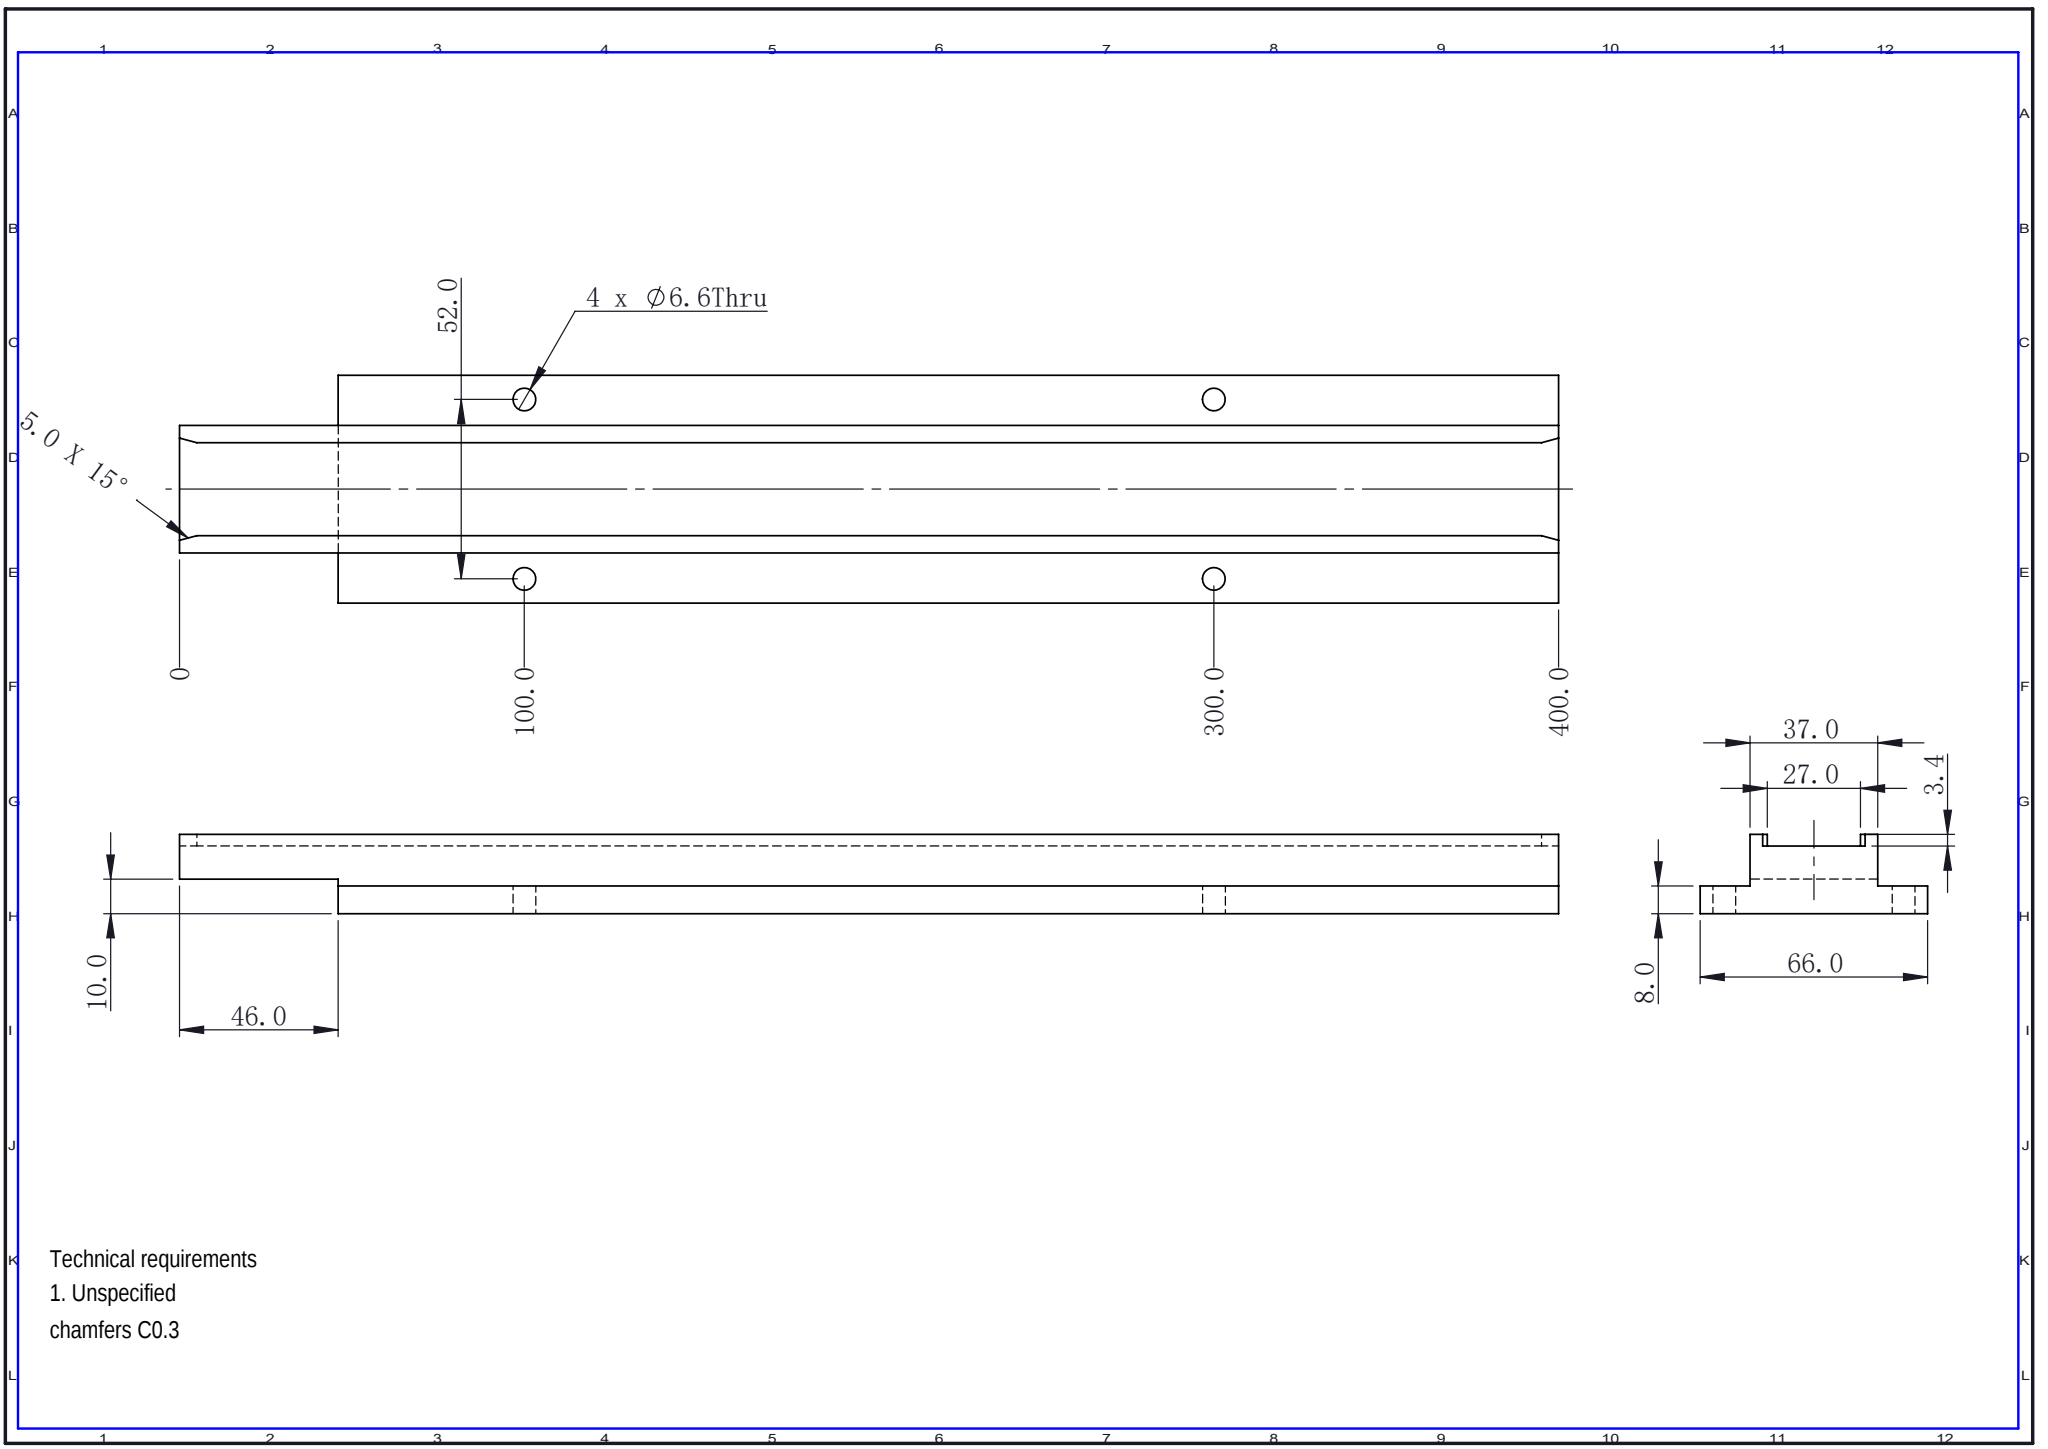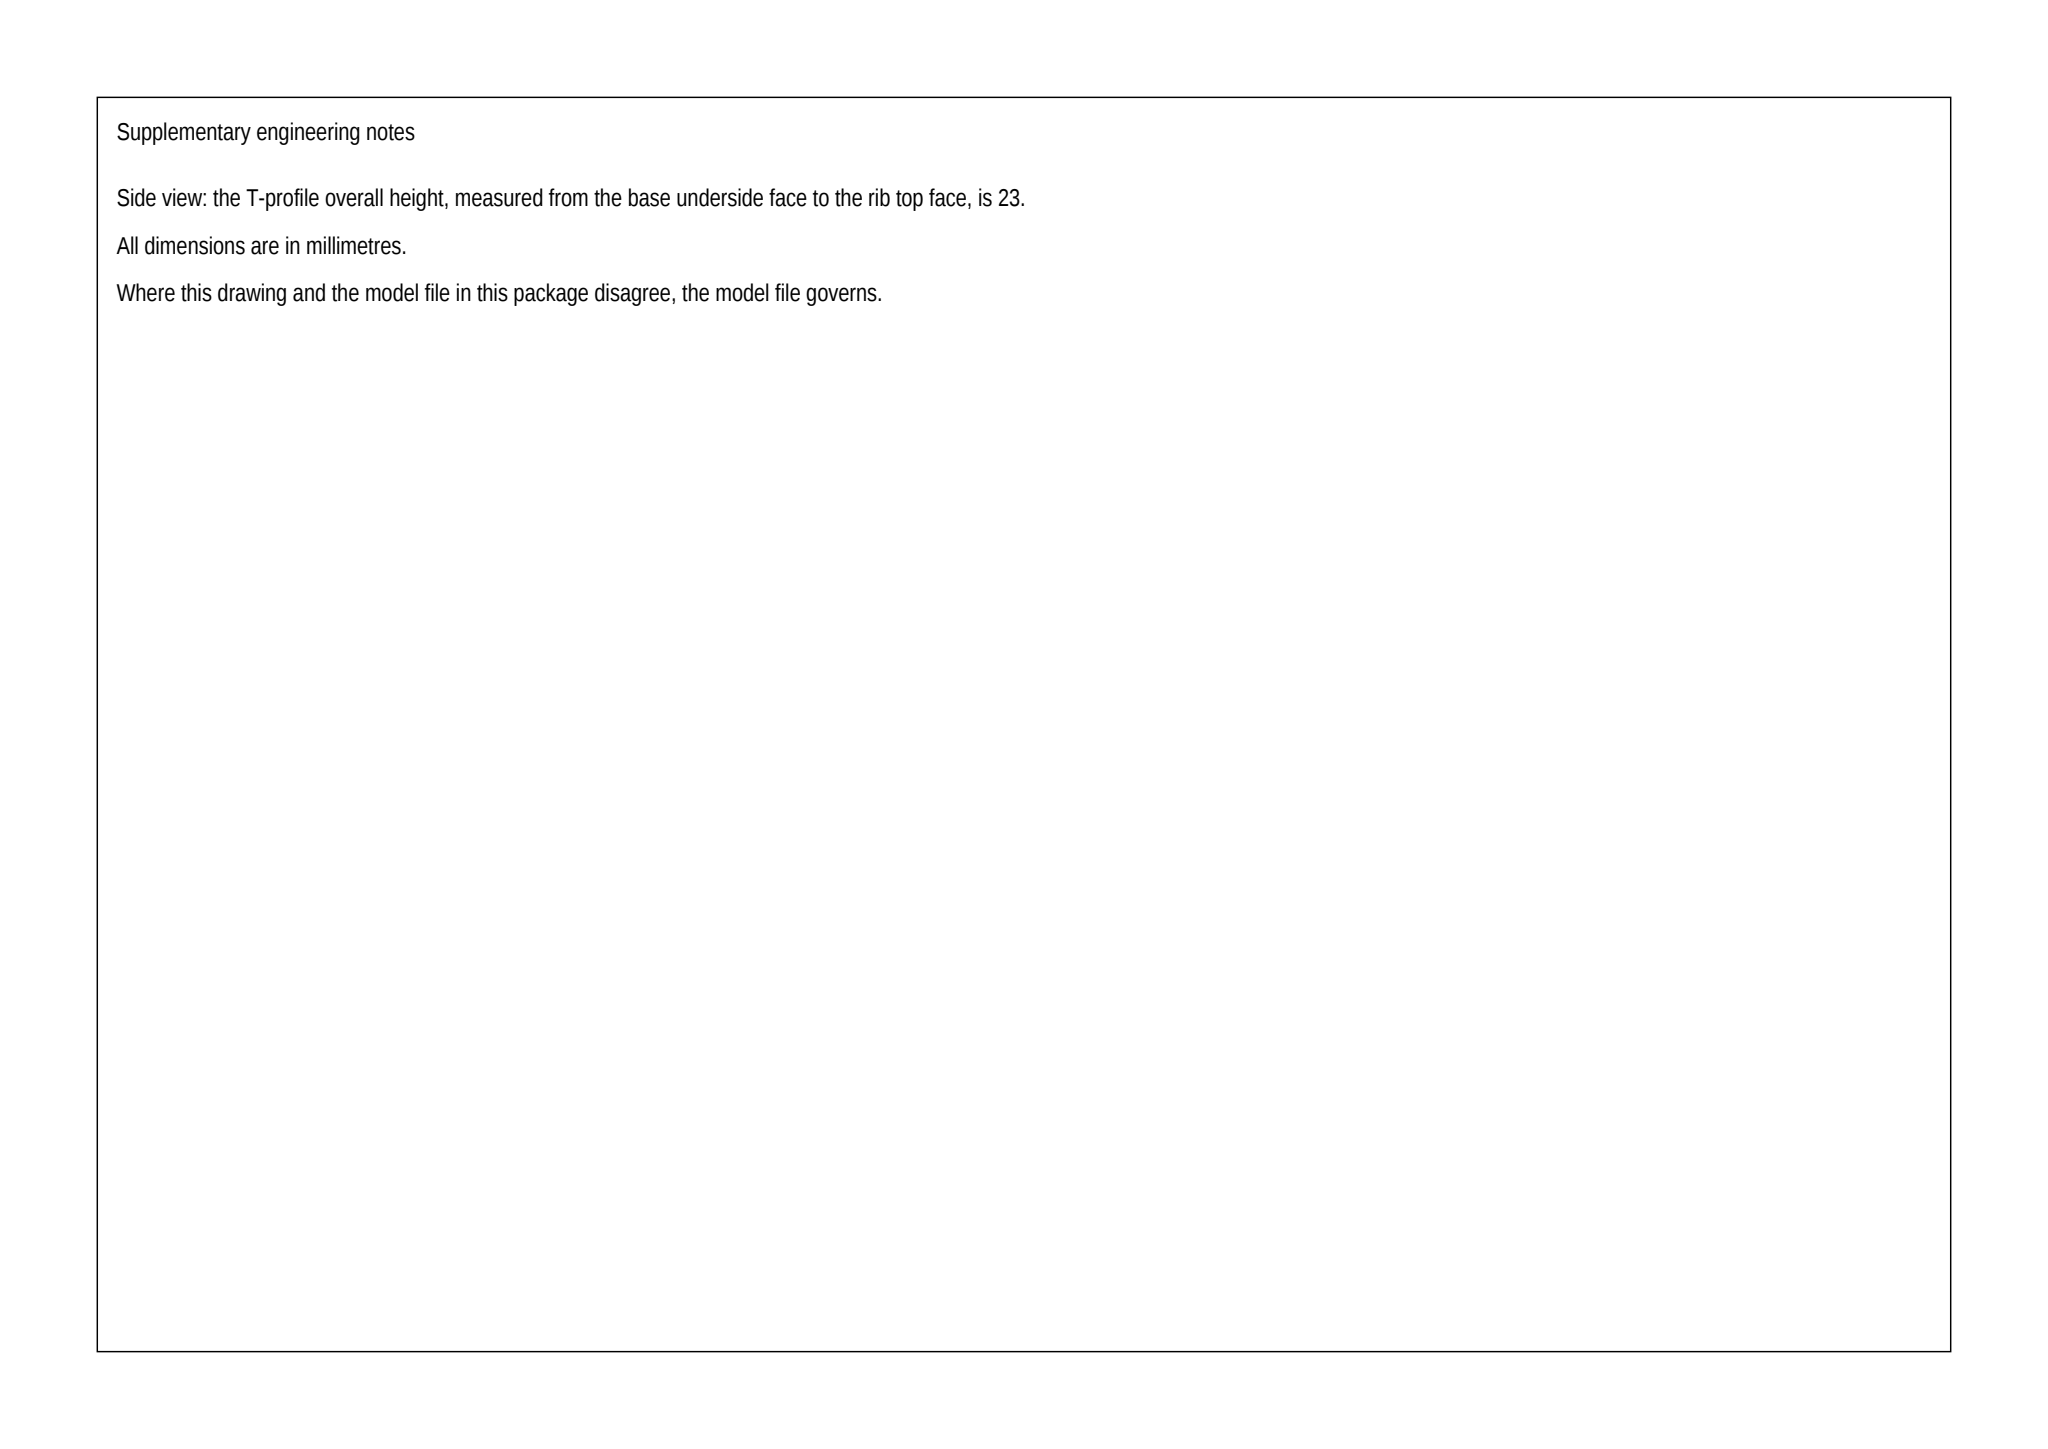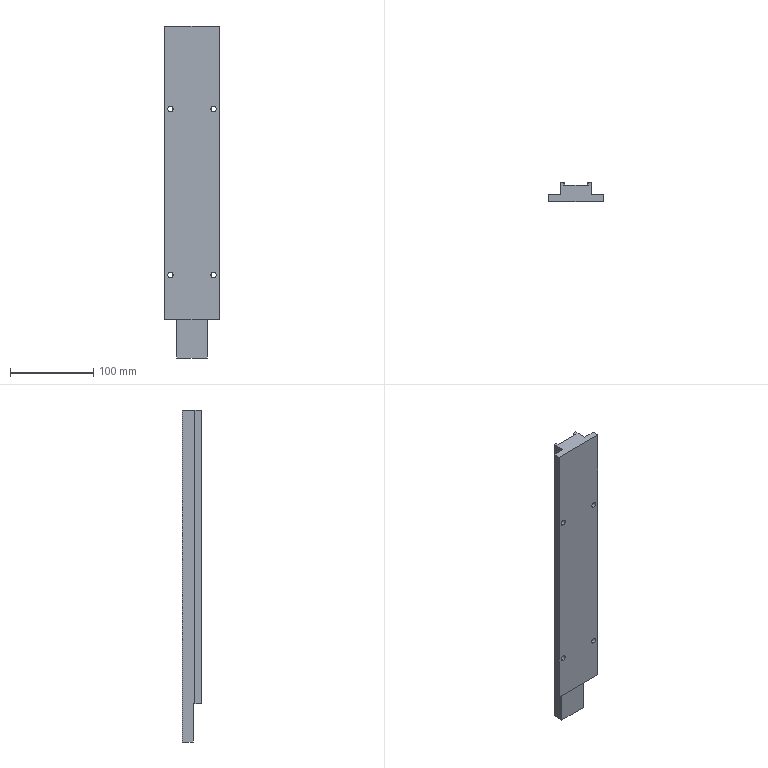Part | SolidWorks | mm | 1 solid | 28 faces | box 66 x 23 x 400 mm | volume 367648 mm3 | plane 20 | cylinder 8 | commonest cylinder face diameters 6.6 x8
build123d program:
from build123d import *
from OCP.BRepFilletAPI import BRepFilletAPI_MakeChamfer

# Parameters (mm, degrees)
BOSS_EXTRUDE1_DEPTH  = 400
SKETCH2_W            = 14.5
SKETCH2_H            = 46
CUT_EXTRUDE1_DEPTH   = 406.686
SKETCH3_W            = 46
SKETCH3_H            = 10
CUT_EXTRUDE2_DEPTH   = 404.957
SKETCH4_W            = 27
SKETCH4_H            = 3.4
CUT_EXTRUDE3_DEPTH   = 407.06
CHAMFER1_SIZE        = 5
CHAMFER1_SIZE2       = 1.34
M6_CLEARANCE_HOLE1_D = 6.6


with BuildPart() as part:
    # Sketch1 → Boss-Extrude1 (new body)
    with BuildSketch(Plane.XY):
        Polygon((0, 0), (66, 0), (66, 8), (51.5, 8), (51.5, 23), (14.5, 23), (14.5, 8), (0, 8), align=None)
    extrude(amount=BOSS_EXTRUDE1_DEPTH)

    # Sketch2 → Cut-Extrude1 (cut, through all)
    with BuildSketch(Plane(origin=(0, 8, 0), x_dir=(1, 0, 0), z_dir=(0, 1, 0))):
        with Locations((7.25, -23)):
            Rectangle(SKETCH2_W, SKETCH2_H)
        with Locations((58.75, -23)):
            Rectangle(SKETCH2_W, SKETCH2_H)
    extrude(amount=-CUT_EXTRUDE1_DEPTH, mode=Mode.SUBTRACT)

    # Sketch3 → Cut-Extrude2 (cut, through all)
    with BuildSketch(Plane.ZY.offset(-14.5)):
        with Locations((23, 5)):
            Rectangle(SKETCH3_W, SKETCH3_H)
    extrude(amount=-CUT_EXTRUDE2_DEPTH, mode=Mode.SUBTRACT)

    # Sketch4 → Cut-Extrude3 (cut, through all)
    with BuildSketch(Plane.XY.offset(400)):
        with Locations((33, 21.3)):
            Rectangle(SKETCH4_W, SKETCH4_H)
    extrude(amount=-CUT_EXTRUDE3_DEPTH, mode=Mode.SUBTRACT)

    # Chamfer1: one chamfer whose edges measure the first distance from different faces: ONE call of the kernel's chamfer builder (chamfer() names one face for all edges)
    chamfer1_edges_1 = [part.edges().sort_by_distance(p)[0] for p in [
        (19.5, 21.3, 0),
        (19.5, 21.3, 400),
    ]]
    chamfer1_side_1 = [part.faces().sort_by_distance(p)[0] for p in [
        (19.5, 21.3, 200),
    ]]
    chamfer1_edges_2 = [part.edges().sort_by_distance(p)[0] for p in [
        (46.5, 21.3, 0),
        (46.5, 21.3, 400),
    ]]
    chamfer1_side_2 = [part.faces().sort_by_distance(p)[0] for p in [
        (46.5, 21.3, 200),
    ]]
    chamfer1 = BRepFilletAPI_MakeChamfer(part.part.solid().wrapped)
    for e in chamfer1_edges_1:
        chamfer1.Add(CHAMFER1_SIZE, CHAMFER1_SIZE2, e.wrapped, chamfer1_side_1[0].wrapped)  # the first distance lies on this face
    for e in chamfer1_edges_2:
        chamfer1.Add(CHAMFER1_SIZE, CHAMFER1_SIZE2, e.wrapped, chamfer1_side_2[0].wrapped)  # the first distance lies on this face
    add(Compound.cast(chamfer1.Shape()), mode=Mode.REPLACE)

    # M6 Clearance Hole1 (through all)
    with Locations(Plane(origin=(0, 0, 0), x_dir=(-1, 0, 0), z_dir=(0, -1, 0))):
        with Locations((-7, -100), (-7, -300), (-59, -100), (-59, -300)):
            Hole(M6_CLEARANCE_HOLE1_D / 2)


solid = part.part
STEP:
#1=CARTESIAN_POINT('',(7.,8.,103.3));
#2=VERTEX_POINT('',#1);
#3=CARTESIAN_POINT('',(7.,8.,96.7));
#4=VERTEX_POINT('',#3);
#5=CARTESIAN_POINT('',(7.,8.,100.));
#6=DIRECTION('',(0.,-1.,0.));
#7=DIRECTION('',(0.,0.,-1.));
#8=AXIS2_PLACEMENT_3D('',#5,#6,#7);
#9=CIRCLE('',#8,3.3);
#10=EDGE_CURVE('',#2,#4,#9,.T.);
#11=ORIENTED_EDGE('',*,*,#10,.F.);
#12=CARTESIAN_POINT('',(7.,-0.,103.3));
#13=VERTEX_POINT('',#12);
#14=CARTESIAN_POINT('',(7.,0.,103.3));
#15=DIRECTION('',(0.,-1.,0.));
#16=VECTOR('',#15,1000.);
#17=LINE('',#14,#16);
#18=EDGE_CURVE('',#2,#13,#17,.T.);
#19=ORIENTED_EDGE('',*,*,#18,.T.);
#20=CARTESIAN_POINT('',(7.,-0.,96.7));
#21=VERTEX_POINT('',#20);
#22=CARTESIAN_POINT('',(7.,-0.,100.));
#23=DIRECTION('',(0.,-1.,0.));
#24=DIRECTION('',(0.,0.,-1.));
#25=AXIS2_PLACEMENT_3D('',#22,#23,#24);
#26=CIRCLE('',#25,3.3);
#27=EDGE_CURVE('',#13,#21,#26,.T.);
#28=ORIENTED_EDGE('',*,*,#27,.T.);
#29=CARTESIAN_POINT('',(7.,0.,96.7));
#30=DIRECTION('',(0.,-1.,0.));
#31=VECTOR('',#30,1000.);
#32=LINE('',#29,#31);
#33=EDGE_CURVE('',#4,#21,#32,.T.);
#34=ORIENTED_EDGE('',*,*,#33,.F.);
#35=EDGE_LOOP('',(#11,#19,#28,#34));
#36=FACE_OUTER_BOUND('',#35,.T.);
#37=CARTESIAN_POINT('',(7.,0.,100.));
#38=DIRECTION('',(0.,-1.,0.));
#39=DIRECTION('',(0.,0.,-1.));
#40=AXIS2_PLACEMENT_3D('',#37,#38,#39);
#41=CYLINDRICAL_SURFACE('',#40,3.3);
#42=ADVANCED_FACE('',(#36),#41,.F.);
#43=CARTESIAN_POINT('',(7.,8.,303.3));
#44=VERTEX_POINT('',#43);
#45=CARTESIAN_POINT('',(7.,8.,296.7));
#46=VERTEX_POINT('',#45);
#47=CARTESIAN_POINT('',(7.,8.,300.));
#48=DIRECTION('',(0.,-1.,0.));
#49=DIRECTION('',(0.,0.,-1.));
#50=AXIS2_PLACEMENT_3D('',#47,#48,#49);
#51=CIRCLE('',#50,3.3);
#52=EDGE_CURVE('',#44,#46,#51,.T.);
#53=ORIENTED_EDGE('',*,*,#52,.F.);
#54=CARTESIAN_POINT('',(7.,-0.,303.3));
#55=VERTEX_POINT('',#54);
#56=CARTESIAN_POINT('',(7.,0.,303.3));
#57=DIRECTION('',(0.,-1.,0.));
#58=VECTOR('',#57,1000.);
#59=LINE('',#56,#58);
#60=EDGE_CURVE('',#44,#55,#59,.T.);
#61=ORIENTED_EDGE('',*,*,#60,.T.);
#62=CARTESIAN_POINT('',(7.,-0.,296.7));
#63=VERTEX_POINT('',#62);
#64=CARTESIAN_POINT('',(7.,-0.,300.));
#65=DIRECTION('',(0.,-1.,0.));
#66=DIRECTION('',(0.,0.,-1.));
#67=AXIS2_PLACEMENT_3D('',#64,#65,#66);
#68=CIRCLE('',#67,3.3);
#69=EDGE_CURVE('',#55,#63,#68,.T.);
#70=ORIENTED_EDGE('',*,*,#69,.T.);
#71=CARTESIAN_POINT('',(7.,0.,296.7));
#72=DIRECTION('',(0.,-1.,0.));
#73=VECTOR('',#72,1000.);
#74=LINE('',#71,#73);
#75=EDGE_CURVE('',#46,#63,#74,.T.);
#76=ORIENTED_EDGE('',*,*,#75,.F.);
#77=EDGE_LOOP('',(#53,#61,#70,#76));
#78=FACE_OUTER_BOUND('',#77,.T.);
#79=CARTESIAN_POINT('',(7.,0.,300.));
#80=DIRECTION('',(0.,-1.,0.));
#81=DIRECTION('',(0.,0.,-1.));
#82=AXIS2_PLACEMENT_3D('',#79,#80,#81);
#83=CYLINDRICAL_SURFACE('',#82,3.3);
#84=ADVANCED_FACE('',(#78),#83,.F.);
#85=CARTESIAN_POINT('',(59.,8.,103.3));
#86=VERTEX_POINT('',#85);
#87=CARTESIAN_POINT('',(59.,8.,96.7));
#88=VERTEX_POINT('',#87);
#89=CARTESIAN_POINT('',(59.,8.,100.));
#90=DIRECTION('',(0.,-1.,0.));
#91=DIRECTION('',(0.,0.,-1.));
#92=AXIS2_PLACEMENT_3D('',#89,#90,#91);
#93=CIRCLE('',#92,3.3);
#94=EDGE_CURVE('',#86,#88,#93,.T.);
#95=ORIENTED_EDGE('',*,*,#94,.F.);
#96=CARTESIAN_POINT('',(59.,-0.,103.3));
#97=VERTEX_POINT('',#96);
#98=CARTESIAN_POINT('',(59.,0.,103.3));
#99=DIRECTION('',(0.,-1.,0.));
#100=VECTOR('',#99,1000.);
#101=LINE('',#98,#100);
#102=EDGE_CURVE('',#86,#97,#101,.T.);
#103=ORIENTED_EDGE('',*,*,#102,.T.);
#104=CARTESIAN_POINT('',(59.,-0.,96.7));
#105=VERTEX_POINT('',#104);
#106=CARTESIAN_POINT('',(59.,-0.,100.));
#107=DIRECTION('',(0.,-1.,0.));
#108=DIRECTION('',(0.,0.,-1.));
#109=AXIS2_PLACEMENT_3D('',#106,#107,#108);
#110=CIRCLE('',#109,3.3);
#111=EDGE_CURVE('',#97,#105,#110,.T.);
#112=ORIENTED_EDGE('',*,*,#111,.T.);
#113=CARTESIAN_POINT('',(59.,0.,96.7));
#114=DIRECTION('',(0.,-1.,0.));
#115=VECTOR('',#114,1000.);
#116=LINE('',#113,#115);
#117=EDGE_CURVE('',#88,#105,#116,.T.);
#118=ORIENTED_EDGE('',*,*,#117,.F.);
#119=EDGE_LOOP('',(#95,#103,#112,#118));
#120=FACE_OUTER_BOUND('',#119,.T.);
#121=CARTESIAN_POINT('',(59.,0.,100.));
#122=DIRECTION('',(0.,-1.,0.));
#123=DIRECTION('',(0.,0.,-1.));
#124=AXIS2_PLACEMENT_3D('',#121,#122,#123);
#125=CYLINDRICAL_SURFACE('',#124,3.3);
#126=ADVANCED_FACE('',(#120),#125,.F.);
#127=CARTESIAN_POINT('',(59.,8.,303.3));
#128=VERTEX_POINT('',#127);
#129=CARTESIAN_POINT('',(59.,8.,296.7));
#130=VERTEX_POINT('',#129);
#131=CARTESIAN_POINT('',(59.,8.,300.));
#132=DIRECTION('',(0.,-1.,0.));
#133=DIRECTION('',(0.,0.,-1.));
#134=AXIS2_PLACEMENT_3D('',#131,#132,#133);
#135=CIRCLE('',#134,3.3);
#136=EDGE_CURVE('',#128,#130,#135,.T.);
#137=ORIENTED_EDGE('',*,*,#136,.F.);
#138=CARTESIAN_POINT('',(59.,-0.,303.3));
#139=VERTEX_POINT('',#138);
#140=CARTESIAN_POINT('',(59.,0.,303.3));
#141=DIRECTION('',(0.,-1.,0.));
#142=VECTOR('',#141,1000.);
#143=LINE('',#140,#142);
#144=EDGE_CURVE('',#128,#139,#143,.T.);
#145=ORIENTED_EDGE('',*,*,#144,.T.);
#146=CARTESIAN_POINT('',(59.,-0.,296.7));
#147=VERTEX_POINT('',#146);
#148=CARTESIAN_POINT('',(59.,-0.,300.));
#149=DIRECTION('',(0.,-1.,0.));
#150=DIRECTION('',(0.,0.,-1.));
#151=AXIS2_PLACEMENT_3D('',#148,#149,#150);
#152=CIRCLE('',#151,3.3);
#153=EDGE_CURVE('',#139,#147,#152,.T.);
#154=ORIENTED_EDGE('',*,*,#153,.T.);
#155=CARTESIAN_POINT('',(59.,0.,296.7));
#156=DIRECTION('',(0.,-1.,0.));
#157=VECTOR('',#156,1000.);
#158=LINE('',#155,#157);
#159=EDGE_CURVE('',#130,#147,#158,.T.);
#160=ORIENTED_EDGE('',*,*,#159,.F.);
#161=EDGE_LOOP('',(#137,#145,#154,#160));
#162=FACE_OUTER_BOUND('',#161,.T.);
#163=CARTESIAN_POINT('',(59.,0.,300.));
#164=DIRECTION('',(0.,-1.,0.));
#165=DIRECTION('',(0.,0.,-1.));
#166=AXIS2_PLACEMENT_3D('',#163,#164,#165);
#167=CYLINDRICAL_SURFACE('',#166,3.3);
#168=ADVANCED_FACE('',(#162),#167,.F.);
#169=CARTESIAN_POINT('',(19.5,23.,5.));
#170=VERTEX_POINT('',#169);
#171=CARTESIAN_POINT('',(19.5,23.,395.));
#172=VERTEX_POINT('',#171);
#173=CARTESIAN_POINT('',(19.5,23.,0.));
#174=DIRECTION('',(0.,0.,1.));
#175=VECTOR('',#174,1000.);
#176=LINE('',#173,#175);
#177=EDGE_CURVE('',#170,#172,#176,.T.);
#178=ORIENTED_EDGE('',*,*,#177,.F.);
#179=CARTESIAN_POINT('',(18.16,23.,0.));
#180=VERTEX_POINT('',#179);
#181=CARTESIAN_POINT('',(18.16,23.,0.));
#182=DIRECTION('',(-0.2588,0.,-0.9659));
#183=VECTOR('',#182,1000.);
#184=LINE('',#181,#183);
#185=EDGE_CURVE('',#170,#180,#184,.T.);
#186=ORIENTED_EDGE('',*,*,#185,.T.);
#187=CARTESIAN_POINT('',(14.5,23.,0.));
#188=VERTEX_POINT('',#187);
#189=CARTESIAN_POINT('',(14.5,23.,0.));
#190=DIRECTION('',(-1.,0.,0.));
#191=VECTOR('',#190,1000.);
#192=LINE('',#189,#191);
#193=EDGE_CURVE('',#180,#188,#192,.T.);
#194=ORIENTED_EDGE('',*,*,#193,.T.);
#195=CARTESIAN_POINT('',(14.5,23.,400.));
#196=VERTEX_POINT('',#195);
#197=CARTESIAN_POINT('',(14.5,23.,400.));
#198=DIRECTION('',(0.,0.,-1.));
#199=VECTOR('',#198,1000.);
#200=LINE('',#197,#199);
#201=EDGE_CURVE('',#196,#188,#200,.T.);
#202=ORIENTED_EDGE('',*,*,#201,.F.);
#203=CARTESIAN_POINT('',(18.16,23.,400.));
#204=VERTEX_POINT('',#203);
#205=CARTESIAN_POINT('',(14.5,23.,400.));
#206=DIRECTION('',(-1.,0.,0.));
#207=VECTOR('',#206,1000.);
#208=LINE('',#205,#207);
#209=EDGE_CURVE('',#204,#196,#208,.T.);
#210=ORIENTED_EDGE('',*,*,#209,.F.);
#211=CARTESIAN_POINT('',(19.5,23.,395.));
#212=DIRECTION('',(0.2588,0.,-0.9659));
#213=VECTOR('',#212,1000.);
#214=LINE('',#211,#213);
#215=EDGE_CURVE('',#204,#172,#214,.T.);
#216=ORIENTED_EDGE('',*,*,#215,.T.);
#217=EDGE_LOOP('',(#178,#186,#194,#202,#210,#216));
#218=FACE_OUTER_BOUND('',#217,.T.);
#219=CARTESIAN_POINT('',(14.5,23.,400.));
#220=DIRECTION('',(0.,-1.,0.));
#221=DIRECTION('',(0.,0.,-1.));
#222=AXIS2_PLACEMENT_3D('',#219,#220,#221);
#223=PLANE('',#222);
#224=ADVANCED_FACE('',(#218),#223,.F.);
#225=CARTESIAN_POINT('',(0.,8.,400.));
#226=VERTEX_POINT('',#225);
#227=CARTESIAN_POINT('',(0.,8.,46.));
#228=VERTEX_POINT('',#227);
#229=CARTESIAN_POINT('',(0.,8.,400.));
#230=DIRECTION('',(0.,0.,-1.));
#231=VECTOR('',#230,1000.);
#232=LINE('',#229,#231);
#233=EDGE_CURVE('',#226,#228,#232,.T.);
#234=ORIENTED_EDGE('',*,*,#233,.T.);
#235=CARTESIAN_POINT('',(0.,0.,46.));
#236=VERTEX_POINT('',#235);
#237=CARTESIAN_POINT('',(0.,0.,46.));
#238=DIRECTION('',(0.,1.,0.));
#239=VECTOR('',#238,1000.);
#240=LINE('',#237,#239);
#241=EDGE_CURVE('',#236,#228,#240,.T.);
#242=ORIENTED_EDGE('',*,*,#241,.F.);
#243=CARTESIAN_POINT('',(0.,0.,400.));
#244=VERTEX_POINT('',#243);
#245=CARTESIAN_POINT('',(0.,0.,400.));
#246=DIRECTION('',(0.,0.,-1.));
#247=VECTOR('',#246,1000.);
#248=LINE('',#245,#247);
#249=EDGE_CURVE('',#244,#236,#248,.T.);
#250=ORIENTED_EDGE('',*,*,#249,.F.);
#251=CARTESIAN_POINT('',(0.,0.,400.));
#252=DIRECTION('',(0.,-1.,0.));
#253=VECTOR('',#252,1000.);
#254=LINE('',#251,#253);
#255=EDGE_CURVE('',#226,#244,#254,.T.);
#256=ORIENTED_EDGE('',*,*,#255,.F.);
#257=EDGE_LOOP('',(#234,#242,#250,#256));
#258=FACE_OUTER_BOUND('',#257,.T.);
#259=CARTESIAN_POINT('',(0.,0.,400.));
#260=DIRECTION('',(1.,0.,0.));
#261=DIRECTION('',(0.,0.,-1.));
#262=AXIS2_PLACEMENT_3D('',#259,#260,#261);
#263=PLANE('',#262);
#264=ADVANCED_FACE('',(#258),#263,.F.);
#265=CARTESIAN_POINT('',(7.,-0.,100.));
#266=DIRECTION('',(0.,-1.,0.));
#267=DIRECTION('',(0.,0.,-1.));
#268=AXIS2_PLACEMENT_3D('',#265,#266,#267);
#269=CIRCLE('',#268,3.3);
#270=EDGE_CURVE('',#21,#13,#269,.T.);
#271=ORIENTED_EDGE('',*,*,#270,.F.);
#272=ORIENTED_EDGE('',*,*,#27,.F.);
#273=EDGE_LOOP('',(#271,#272));
#274=FACE_BOUND('',#273,.T.);
#275=CARTESIAN_POINT('',(7.,-0.,300.));
#276=DIRECTION('',(0.,-1.,0.));
#277=DIRECTION('',(0.,0.,-1.));
#278=AXIS2_PLACEMENT_3D('',#275,#276,#277);
#279=CIRCLE('',#278,3.3);
#280=EDGE_CURVE('',#63,#55,#279,.T.);
#281=ORIENTED_EDGE('',*,*,#280,.F.);
#282=ORIENTED_EDGE('',*,*,#69,.F.);
#283=EDGE_LOOP('',(#281,#282));
#284=FACE_BOUND('',#283,.T.);
#285=CARTESIAN_POINT('',(59.,-0.,100.));
#286=DIRECTION('',(0.,-1.,0.));
#287=DIRECTION('',(0.,0.,-1.));
#288=AXIS2_PLACEMENT_3D('',#285,#286,#287);
#289=CIRCLE('',#288,3.3);
#290=EDGE_CURVE('',#105,#97,#289,.T.);
#291=ORIENTED_EDGE('',*,*,#290,.F.);
#292=ORIENTED_EDGE('',*,*,#111,.F.);
#293=EDGE_LOOP('',(#291,#292));
#294=FACE_BOUND('',#293,.T.);
#295=CARTESIAN_POINT('',(59.,-0.,300.));
#296=DIRECTION('',(0.,-1.,0.));
#297=DIRECTION('',(0.,0.,-1.));
#298=AXIS2_PLACEMENT_3D('',#295,#296,#297);
#299=CIRCLE('',#298,3.3);
#300=EDGE_CURVE('',#147,#139,#299,.T.);
#301=ORIENTED_EDGE('',*,*,#300,.F.);
#302=ORIENTED_EDGE('',*,*,#153,.F.);
#303=EDGE_LOOP('',(#301,#302));
#304=FACE_BOUND('',#303,.T.);
#305=CARTESIAN_POINT('',(66.,0.,46.));
#306=VERTEX_POINT('',#305);
#307=CARTESIAN_POINT('',(0.,0.,46.));
#308=DIRECTION('',(1.,0.,-0.));
#309=VECTOR('',#308,1000.);
#310=LINE('',#307,#309);
#311=EDGE_CURVE('',#236,#306,#310,.T.);
#312=ORIENTED_EDGE('',*,*,#311,.T.);
#313=CARTESIAN_POINT('',(66.,0.,400.));
#314=VERTEX_POINT('',#313);
#315=CARTESIAN_POINT('',(66.,0.,400.));
#316=DIRECTION('',(0.,0.,-1.));
#317=VECTOR('',#316,1000.);
#318=LINE('',#315,#317);
#319=EDGE_CURVE('',#314,#306,#318,.T.);
#320=ORIENTED_EDGE('',*,*,#319,.F.);
#321=CARTESIAN_POINT('',(0.,0.,400.));
#322=DIRECTION('',(1.,0.,0.));
#323=VECTOR('',#322,1000.);
#324=LINE('',#321,#323);
#325=EDGE_CURVE('',#244,#314,#324,.T.);
#326=ORIENTED_EDGE('',*,*,#325,.F.);
#327=ORIENTED_EDGE('',*,*,#249,.T.);
#328=EDGE_LOOP('',(#312,#320,#326,#327));
#329=FACE_OUTER_BOUND('',#328,.T.);
#330=CARTESIAN_POINT('',(0.,0.,400.));
#331=DIRECTION('',(0.,1.,0.));
#332=DIRECTION('',(0.,0.,1.));
#333=AXIS2_PLACEMENT_3D('',#330,#331,#332);
#334=PLANE('',#333);
#335=ADVANCED_FACE('',(#274,#284,#294,#304,#329),#334,.F.);
#336=ORIENTED_EDGE('',*,*,#319,.T.);
#337=CARTESIAN_POINT('',(66.,8.,46.));
#338=VERTEX_POINT('',#337);
#339=CARTESIAN_POINT('',(66.,0.,46.));
#340=DIRECTION('',(0.,1.,0.));
#341=VECTOR('',#340,1000.);
#342=LINE('',#339,#341);
#343=EDGE_CURVE('',#306,#338,#342,.T.);
#344=ORIENTED_EDGE('',*,*,#343,.T.);
#345=CARTESIAN_POINT('',(66.,8.,400.));
#346=VERTEX_POINT('',#345);
#347=CARTESIAN_POINT('',(66.,8.,400.));
#348=DIRECTION('',(0.,0.,-1.));
#349=VECTOR('',#348,1000.);
#350=LINE('',#347,#349);
#351=EDGE_CURVE('',#346,#338,#350,.T.);
#352=ORIENTED_EDGE('',*,*,#351,.F.);
#353=CARTESIAN_POINT('',(66.,0.,400.));
#354=DIRECTION('',(0.,1.,0.));
#355=VECTOR('',#354,1000.);
#356=LINE('',#353,#355);
#357=EDGE_CURVE('',#314,#346,#356,.T.);
#358=ORIENTED_EDGE('',*,*,#357,.F.);
#359=EDGE_LOOP('',(#336,#344,#352,#358));
#360=FACE_OUTER_BOUND('',#359,.T.);
#361=CARTESIAN_POINT('',(66.,0.,400.));
#362=DIRECTION('',(-1.,0.,0.));
#363=DIRECTION('',(0.,0.,1.));
#364=AXIS2_PLACEMENT_3D('',#361,#362,#363);
#365=PLANE('',#364);
#366=ADVANCED_FACE('',(#360),#365,.F.);
#367=CARTESIAN_POINT('',(59.,8.,100.));
#368=DIRECTION('',(0.,-1.,0.));
#369=DIRECTION('',(0.,0.,-1.));
#370=AXIS2_PLACEMENT_3D('',#367,#368,#369);
#371=CIRCLE('',#370,3.3);
#372=EDGE_CURVE('',#88,#86,#371,.T.);
#373=ORIENTED_EDGE('',*,*,#372,.T.);
#374=ORIENTED_EDGE('',*,*,#94,.T.);
#375=EDGE_LOOP('',(#373,#374));
#376=FACE_BOUND('',#375,.T.);
#377=CARTESIAN_POINT('',(59.,8.,300.));
#378=DIRECTION('',(0.,-1.,0.));
#379=DIRECTION('',(0.,0.,-1.));
#380=AXIS2_PLACEMENT_3D('',#377,#378,#379);
#381=CIRCLE('',#380,3.3);
#382=EDGE_CURVE('',#130,#128,#381,.T.);
#383=ORIENTED_EDGE('',*,*,#382,.T.);
#384=ORIENTED_EDGE('',*,*,#136,.T.);
#385=EDGE_LOOP('',(#383,#384));
#386=FACE_BOUND('',#385,.T.);
#387=ORIENTED_EDGE('',*,*,#351,.T.);
#388=CARTESIAN_POINT('',(51.5,8.,46.));
#389=VERTEX_POINT('',#388);
#390=CARTESIAN_POINT('',(66.,8.,46.));
#391=DIRECTION('',(1.,0.,0.));
#392=VECTOR('',#391,1000.);
#393=LINE('',#390,#392);
#394=EDGE_CURVE('',#389,#338,#393,.T.);
#395=ORIENTED_EDGE('',*,*,#394,.F.);
#396=CARTESIAN_POINT('',(51.5,8.,400.));
#397=VERTEX_POINT('',#396);
#398=CARTESIAN_POINT('',(51.5,8.,400.));
#399=DIRECTION('',(0.,0.,-1.));
#400=VECTOR('',#399,1000.);
#401=LINE('',#398,#400);
#402=EDGE_CURVE('',#397,#389,#401,.T.);
#403=ORIENTED_EDGE('',*,*,#402,.F.);
#404=CARTESIAN_POINT('',(66.,8.,400.));
#405=DIRECTION('',(-1.,0.,0.));
#406=VECTOR('',#405,1000.);
#407=LINE('',#404,#406);
#408=EDGE_CURVE('',#346,#397,#407,.T.);
#409=ORIENTED_EDGE('',*,*,#408,.F.);
#410=EDGE_LOOP('',(#387,#395,#403,#409));
#411=FACE_OUTER_BOUND('',#410,.T.);
#412=CARTESIAN_POINT('',(66.,8.,400.));
#413=DIRECTION('',(0.,-1.,0.));
#414=DIRECTION('',(0.,0.,-1.));
#415=AXIS2_PLACEMENT_3D('',#412,#413,#414);
#416=PLANE('',#415);
#417=ADVANCED_FACE('',(#376,#386,#411),#416,.F.);
#418=CARTESIAN_POINT('',(51.5,10.,46.));
#419=VERTEX_POINT('',#418);
#420=CARTESIAN_POINT('',(51.5,23.,46.));
#421=DIRECTION('',(-0.,1.,0.));
#422=VECTOR('',#421,1000.);
#423=LINE('',#420,#422);
#424=EDGE_CURVE('',#389,#419,#423,.T.);
#425=ORIENTED_EDGE('',*,*,#424,.T.);
#426=CARTESIAN_POINT('',(51.5,10.,0.));
#427=VERTEX_POINT('',#426);
#428=CARTESIAN_POINT('',(51.5,10.,400.));
#429=DIRECTION('',(0.,0.,-1.));
#430=VECTOR('',#429,1000.);
#431=LINE('',#428,#430);
#432=EDGE_CURVE('',#419,#427,#431,.T.);
#433=ORIENTED_EDGE('',*,*,#432,.T.);
#434=CARTESIAN_POINT('',(51.5,23.,0.));
#435=VERTEX_POINT('',#434);
#436=CARTESIAN_POINT('',(51.5,23.,0.));
#437=DIRECTION('',(-0.,1.,0.));
#438=VECTOR('',#437,1000.);
#439=LINE('',#436,#438);
#440=EDGE_CURVE('',#427,#435,#439,.T.);
#441=ORIENTED_EDGE('',*,*,#440,.T.);
#442=CARTESIAN_POINT('',(51.5,23.,400.));
#443=VERTEX_POINT('',#442);
#444=CARTESIAN_POINT('',(51.5,23.,400.));
#445=DIRECTION('',(0.,0.,-1.));
#446=VECTOR('',#445,1000.);
#447=LINE('',#444,#446);
#448=EDGE_CURVE('',#443,#435,#447,.T.);
#449=ORIENTED_EDGE('',*,*,#448,.F.);
#450=CARTESIAN_POINT('',(51.5,23.,400.));
#451=DIRECTION('',(-0.,1.,0.));
#452=VECTOR('',#451,1000.);
#453=LINE('',#450,#452);
#454=EDGE_CURVE('',#397,#443,#453,.T.);
#455=ORIENTED_EDGE('',*,*,#454,.F.);
#456=ORIENTED_EDGE('',*,*,#402,.T.);
#457=EDGE_LOOP('',(#425,#433,#441,#449,#455,#456));
#458=FACE_OUTER_BOUND('',#457,.T.);
#459=CARTESIAN_POINT('',(51.5,23.,400.));
#460=DIRECTION('',(-1.,-0.,0.));
#461=DIRECTION('',(0.,-1.,0.));
#462=AXIS2_PLACEMENT_3D('',#459,#460,#461);
#463=PLANE('',#462);
#464=ADVANCED_FACE('',(#458),#463,.F.);
#465=CARTESIAN_POINT('',(47.84,23.,0.));
#466=VERTEX_POINT('',#465);
#467=CARTESIAN_POINT('',(14.5,23.,0.));
#468=DIRECTION('',(-1.,0.,0.));
#469=VECTOR('',#468,1000.);
#470=LINE('',#467,#469);
#471=EDGE_CURVE('',#435,#466,#470,.T.);
#472=ORIENTED_EDGE('',*,*,#471,.T.);
#473=CARTESIAN_POINT('',(46.5,23.,5.));
#474=VERTEX_POINT('',#473);
#475=CARTESIAN_POINT('',(47.84,23.,0.));
#476=DIRECTION('',(-0.2588,0.,0.9659));
#477=VECTOR('',#476,1000.);
#478=LINE('',#475,#477);
#479=EDGE_CURVE('',#466,#474,#478,.T.);
#480=ORIENTED_EDGE('',*,*,#479,.T.);
#481=CARTESIAN_POINT('',(46.5,23.,395.));
#482=VERTEX_POINT('',#481);
#483=CARTESIAN_POINT('',(46.5,23.,0.));
#484=DIRECTION('',(0.,0.,1.));
#485=VECTOR('',#484,1000.);
#486=LINE('',#483,#485);
#487=EDGE_CURVE('',#474,#482,#486,.T.);
#488=ORIENTED_EDGE('',*,*,#487,.T.);
#489=CARTESIAN_POINT('',(47.84,23.,400.));
#490=VERTEX_POINT('',#489);
#491=CARTESIAN_POINT('',(46.5,23.,395.));
#492=DIRECTION('',(0.2588,0.,0.9659));
#493=VECTOR('',#492,1000.);
#494=LINE('',#491,#493);
#495=EDGE_CURVE('',#482,#490,#494,.T.);
#496=ORIENTED_EDGE('',*,*,#495,.T.);
#497=CARTESIAN_POINT('',(14.5,23.,400.));
#498=DIRECTION('',(-1.,0.,0.));
#499=VECTOR('',#498,1000.);
#500=LINE('',#497,#499);
#501=EDGE_CURVE('',#443,#490,#500,.T.);
#502=ORIENTED_EDGE('',*,*,#501,.F.);
#503=ORIENTED_EDGE('',*,*,#448,.T.);
#504=EDGE_LOOP('',(#472,#480,#488,#496,#502,#503));
#505=FACE_OUTER_BOUND('',#504,.T.);
#506=CARTESIAN_POINT('',(14.5,23.,400.));
#507=DIRECTION('',(0.,-1.,0.));
#508=DIRECTION('',(0.,0.,-1.));
#509=AXIS2_PLACEMENT_3D('',#506,#507,#508);
#510=PLANE('',#509);
#511=ADVANCED_FACE('',(#505),#510,.F.);
#512=CARTESIAN_POINT('',(14.5,10.,0.));
#513=VERTEX_POINT('',#512);
#514=CARTESIAN_POINT('',(14.5,23.,0.));
#515=DIRECTION('',(0.,-1.,0.));
#516=VECTOR('',#515,1000.);
#517=LINE('',#514,#516);
#518=EDGE_CURVE('',#188,#513,#517,.T.);
#519=ORIENTED_EDGE('',*,*,#518,.T.);
#520=CARTESIAN_POINT('',(14.5,10.,46.));
#521=VERTEX_POINT('',#520);
#522=CARTESIAN_POINT('',(14.5,10.,0.));
#523=DIRECTION('',(0.,0.,-1.));
#524=VECTOR('',#523,1000.);
#525=LINE('',#522,#524);
#526=EDGE_CURVE('',#521,#513,#525,.T.);
#527=ORIENTED_EDGE('',*,*,#526,.F.);
#528=CARTESIAN_POINT('',(14.5,8.,46.));
#529=VERTEX_POINT('',#528);
#530=CARTESIAN_POINT('',(14.5,0.,46.));
#531=DIRECTION('',(-0.,1.,0.));
#532=VECTOR('',#531,1000.);
#533=LINE('',#530,#532);
#534=EDGE_CURVE('',#529,#521,#533,.T.);
#535=ORIENTED_EDGE('',*,*,#534,.F.);
#536=CARTESIAN_POINT('',(14.5,8.,400.));
#537=VERTEX_POINT('',#536);
#538=CARTESIAN_POINT('',(14.5,8.,400.));
#539=DIRECTION('',(0.,0.,-1.));
#540=VECTOR('',#539,1000.);
#541=LINE('',#538,#540);
#542=EDGE_CURVE('',#537,#529,#541,.T.);
#543=ORIENTED_EDGE('',*,*,#542,.F.);
#544=CARTESIAN_POINT('',(14.5,23.,400.));
#545=DIRECTION('',(0.,-1.,0.));
#546=VECTOR('',#545,1000.);
#547=LINE('',#544,#546);
#548=EDGE_CURVE('',#196,#537,#547,.T.);
#549=ORIENTED_EDGE('',*,*,#548,.F.);
#550=ORIENTED_EDGE('',*,*,#201,.T.);
#551=EDGE_LOOP('',(#519,#527,#535,#543,#549,#550));
#552=FACE_OUTER_BOUND('',#551,.T.);
#553=CARTESIAN_POINT('',(14.5,23.,400.));
#554=DIRECTION('',(1.,0.,0.));
#555=DIRECTION('',(-0.,1.,0.));
#556=AXIS2_PLACEMENT_3D('',#553,#554,#555);
#557=PLANE('',#556);
#558=ADVANCED_FACE('',(#552),#557,.F.);
#559=CARTESIAN_POINT('',(7.,8.,100.));
#560=DIRECTION('',(0.,-1.,0.));
#561=DIRECTION('',(0.,0.,-1.));
#562=AXIS2_PLACEMENT_3D('',#559,#560,#561);
#563=CIRCLE('',#562,3.3);
#564=EDGE_CURVE('',#4,#2,#563,.T.);
#565=ORIENTED_EDGE('',*,*,#564,.T.);
#566=ORIENTED_EDGE('',*,*,#10,.T.);
#567=EDGE_LOOP('',(#565,#566));
#568=FACE_BOUND('',#567,.T.);
#569=CARTESIAN_POINT('',(7.,8.,300.));
#570=DIRECTION('',(0.,-1.,0.));
#571=DIRECTION('',(0.,0.,-1.));
#572=AXIS2_PLACEMENT_3D('',#569,#570,#571);
#573=CIRCLE('',#572,3.3);
#574=EDGE_CURVE('',#46,#44,#573,.T.);
#575=ORIENTED_EDGE('',*,*,#574,.T.);
#576=ORIENTED_EDGE('',*,*,#52,.T.);
#577=EDGE_LOOP('',(#575,#576));
#578=FACE_BOUND('',#577,.T.);
#579=ORIENTED_EDGE('',*,*,#542,.T.);
#580=CARTESIAN_POINT('',(0.,8.,46.));
#581=DIRECTION('',(1.,0.,-0.));
#582=VECTOR('',#581,1000.);
#583=LINE('',#580,#582);
#584=EDGE_CURVE('',#228,#529,#583,.T.);
#585=ORIENTED_EDGE('',*,*,#584,.F.);
#586=ORIENTED_EDGE('',*,*,#233,.F.);
#587=CARTESIAN_POINT('',(0.,8.,400.));
#588=DIRECTION('',(-1.,0.,0.));
#589=VECTOR('',#588,1000.);
#590=LINE('',#587,#589);
#591=EDGE_CURVE('',#537,#226,#590,.T.);
#592=ORIENTED_EDGE('',*,*,#591,.F.);
#593=EDGE_LOOP('',(#579,#585,#586,#592));
#594=FACE_OUTER_BOUND('',#593,.T.);
#595=CARTESIAN_POINT('',(0.,8.,400.));
#596=DIRECTION('',(0.,-1.,0.));
#597=DIRECTION('',(0.,0.,-1.));
#598=AXIS2_PLACEMENT_3D('',#595,#596,#597);
#599=PLANE('',#598);
#600=ADVANCED_FACE('',(#568,#578,#594),#599,.F.);
#601=CARTESIAN_POINT('',(18.16,19.6,400.));
#602=VERTEX_POINT('',#601);
#603=CARTESIAN_POINT('',(47.84,19.6,400.));
#604=VERTEX_POINT('',#603);
#605=CARTESIAN_POINT('',(19.5,19.6,400.));
#606=DIRECTION('',(1.,0.,0.));
#607=VECTOR('',#606,1000.);
#608=LINE('',#605,#607);
#609=EDGE_CURVE('',#602,#604,#608,.T.);
#610=ORIENTED_EDGE('',*,*,#609,.F.);
#611=CARTESIAN_POINT('',(18.16,0.,400.));
#612=DIRECTION('',(0.,1.,0.));
#613=VECTOR('',#612,1000.);
#614=LINE('',#611,#613);
#615=EDGE_CURVE('',#602,#204,#614,.T.);
#616=ORIENTED_EDGE('',*,*,#615,.T.);
#617=ORIENTED_EDGE('',*,*,#209,.T.);
#618=ORIENTED_EDGE('',*,*,#548,.T.);
#619=ORIENTED_EDGE('',*,*,#591,.T.);
#620=ORIENTED_EDGE('',*,*,#255,.T.);
#621=ORIENTED_EDGE('',*,*,#325,.T.);
#622=ORIENTED_EDGE('',*,*,#357,.T.);
#623=ORIENTED_EDGE('',*,*,#408,.T.);
#624=ORIENTED_EDGE('',*,*,#454,.T.);
#625=ORIENTED_EDGE('',*,*,#501,.T.);
#626=CARTESIAN_POINT('',(47.84,0.,400.));
#627=DIRECTION('',(0.,-1.,0.));
#628=VECTOR('',#627,1000.);
#629=LINE('',#626,#628);
#630=EDGE_CURVE('',#490,#604,#629,.T.);
#631=ORIENTED_EDGE('',*,*,#630,.T.);
#632=EDGE_LOOP('',(#610,#616,#617,#618,#619,#620,#621,#622,#623,#624,#625,#631));
#633=FACE_OUTER_BOUND('',#632,.T.);
#634=CARTESIAN_POINT('',(0.,0.,400.));
#635=DIRECTION('',(0.,0.,-1.));
#636=DIRECTION('',(-1.,0.,0.));
#637=AXIS2_PLACEMENT_3D('',#634,#635,#636);
#638=PLANE('',#637);
#639=ADVANCED_FACE('',(#633),#638,.F.);
#640=ORIENTED_EDGE('',*,*,#193,.F.);
#641=CARTESIAN_POINT('',(18.16,19.6,0.));
#642=VERTEX_POINT('',#641);
#643=CARTESIAN_POINT('',(18.16,19.6,0.));
#644=DIRECTION('',(0.,-1.,0.));
#645=VECTOR('',#644,1000.);
#646=LINE('',#643,#645);
#647=EDGE_CURVE('',#180,#642,#646,.T.);
#648=ORIENTED_EDGE('',*,*,#647,.T.);
#649=CARTESIAN_POINT('',(47.84,19.6,0.));
#650=VERTEX_POINT('',#649);
#651=CARTESIAN_POINT('',(19.5,19.6,0.));
#652=DIRECTION('',(1.,0.,0.));
#653=VECTOR('',#652,1000.);
#654=LINE('',#651,#653);
#655=EDGE_CURVE('',#642,#650,#654,.T.);
#656=ORIENTED_EDGE('',*,*,#655,.T.);
#657=CARTESIAN_POINT('',(47.84,23.,0.));
#658=DIRECTION('',(0.,1.,0.));
#659=VECTOR('',#658,1000.);
#660=LINE('',#657,#659);
#661=EDGE_CURVE('',#650,#466,#660,.T.);
#662=ORIENTED_EDGE('',*,*,#661,.T.);
#663=ORIENTED_EDGE('',*,*,#471,.F.);
#664=ORIENTED_EDGE('',*,*,#440,.F.);
#665=CARTESIAN_POINT('',(-0.,10.,0.));
#666=DIRECTION('',(1.,0.,0.));
#667=VECTOR('',#666,1000.);
#668=LINE('',#665,#667);
#669=EDGE_CURVE('',#513,#427,#668,.T.);
#670=ORIENTED_EDGE('',*,*,#669,.F.);
#671=ORIENTED_EDGE('',*,*,#518,.F.);
#672=EDGE_LOOP('',(#640,#648,#656,#662,#663,#664,#670,#671));
#673=FACE_OUTER_BOUND('',#672,.T.);
#674=CARTESIAN_POINT('',(0.,0.,0.));
#675=DIRECTION('',(0.,0.,-1.));
#676=DIRECTION('',(-1.,0.,0.));
#677=AXIS2_PLACEMENT_3D('',#674,#675,#676);
#678=PLANE('',#677);
#679=ADVANCED_FACE('',(#673),#678,.T.);
#680=ORIENTED_EDGE('',*,*,#584,.T.);
#681=ORIENTED_EDGE('',*,*,#534,.T.);
#682=CARTESIAN_POINT('',(66.,10.,46.));
#683=DIRECTION('',(-1.,-0.,0.));
#684=VECTOR('',#683,1000.);
#685=LINE('',#682,#684);
#686=EDGE_CURVE('',#419,#521,#685,.T.);
#687=ORIENTED_EDGE('',*,*,#686,.F.);
#688=ORIENTED_EDGE('',*,*,#424,.F.);
#689=ORIENTED_EDGE('',*,*,#394,.T.);
#690=ORIENTED_EDGE('',*,*,#343,.F.);
#691=ORIENTED_EDGE('',*,*,#311,.F.);
#692=ORIENTED_EDGE('',*,*,#241,.T.);
#693=EDGE_LOOP('',(#680,#681,#687,#688,#689,#690,#691,#692));
#694=FACE_OUTER_BOUND('',#693,.T.);
#695=CARTESIAN_POINT('',(0.,0.,46.));
#696=DIRECTION('',(0.,0.,1.));
#697=DIRECTION('',(1.,0.,-0.));
#698=AXIS2_PLACEMENT_3D('',#695,#696,#697);
#699=PLANE('',#698);
#700=ADVANCED_FACE('',(#694),#699,.F.);
#701=ORIENTED_EDGE('',*,*,#686,.T.);
#702=ORIENTED_EDGE('',*,*,#526,.T.);
#703=ORIENTED_EDGE('',*,*,#669,.T.);
#704=ORIENTED_EDGE('',*,*,#432,.F.);
#705=EDGE_LOOP('',(#701,#702,#703,#704));
#706=FACE_OUTER_BOUND('',#705,.T.);
#707=CARTESIAN_POINT('',(66.,10.,0.));
#708=DIRECTION('',(-0.,1.,0.));
#709=DIRECTION('',(-1.,-0.,0.));
#710=AXIS2_PLACEMENT_3D('',#707,#708,#709);
#711=PLANE('',#710);
#712=ADVANCED_FACE('',(#706),#711,.F.);
#713=CARTESIAN_POINT('',(19.5,19.6,5.));
#714=VERTEX_POINT('',#713);
#715=CARTESIAN_POINT('',(19.5,19.6,395.));
#716=VERTEX_POINT('',#715);
#717=CARTESIAN_POINT('',(19.5,19.6,0.));
#718=DIRECTION('',(0.,0.,1.));
#719=VECTOR('',#718,1000.);
#720=LINE('',#717,#719);
#721=EDGE_CURVE('',#714,#716,#720,.T.);
#722=ORIENTED_EDGE('',*,*,#721,.F.);
#723=CARTESIAN_POINT('',(19.5,23.,5.));
#724=DIRECTION('',(0.,1.,0.));
#725=VECTOR('',#724,1000.);
#726=LINE('',#723,#725);
#727=EDGE_CURVE('',#714,#170,#726,.T.);
#728=ORIENTED_EDGE('',*,*,#727,.T.);
#729=ORIENTED_EDGE('',*,*,#177,.T.);
#730=CARTESIAN_POINT('',(19.5,23.,395.));
#731=DIRECTION('',(0.,-1.,0.));
#732=VECTOR('',#731,1000.);
#733=LINE('',#730,#732);
#734=EDGE_CURVE('',#172,#716,#733,.T.);
#735=ORIENTED_EDGE('',*,*,#734,.T.);
#736=EDGE_LOOP('',(#722,#728,#729,#735));
#737=FACE_OUTER_BOUND('',#736,.T.);
#738=CARTESIAN_POINT('',(19.5,23.,0.));
#739=DIRECTION('',(-1.,0.,0.));
#740=DIRECTION('',(0.,0.,1.));
#741=AXIS2_PLACEMENT_3D('',#738,#739,#740);
#742=PLANE('',#741);
#743=ADVANCED_FACE('',(#737),#742,.F.);
#744=ORIENTED_EDGE('',*,*,#487,.F.);
#745=CARTESIAN_POINT('',(46.5,19.6,5.));
#746=VERTEX_POINT('',#745);
#747=CARTESIAN_POINT('',(46.5,19.6,5.));
#748=DIRECTION('',(0.,-1.,0.));
#749=VECTOR('',#748,1000.);
#750=LINE('',#747,#749);
#751=EDGE_CURVE('',#474,#746,#750,.T.);
#752=ORIENTED_EDGE('',*,*,#751,.T.);
#753=CARTESIAN_POINT('',(46.5,19.6,395.));
#754=VERTEX_POINT('',#753);
#755=CARTESIAN_POINT('',(46.5,19.6,0.));
#756=DIRECTION('',(0.,0.,1.));
#757=VECTOR('',#756,1000.);
#758=LINE('',#755,#757);
#759=EDGE_CURVE('',#746,#754,#758,.T.);
#760=ORIENTED_EDGE('',*,*,#759,.T.);
#761=CARTESIAN_POINT('',(46.5,23.,395.));
#762=DIRECTION('',(0.,1.,0.));
#763=VECTOR('',#762,1000.);
#764=LINE('',#761,#763);
#765=EDGE_CURVE('',#754,#482,#764,.T.);
#766=ORIENTED_EDGE('',*,*,#765,.T.);
#767=EDGE_LOOP('',(#744,#752,#760,#766));
#768=FACE_OUTER_BOUND('',#767,.T.);
#769=CARTESIAN_POINT('',(46.5,23.,0.));
#770=DIRECTION('',(1.,0.,0.));
#771=DIRECTION('',(0.,0.,-1.));
#772=AXIS2_PLACEMENT_3D('',#769,#770,#771);
#773=PLANE('',#772);
#774=ADVANCED_FACE('',(#768),#773,.F.);
#775=ORIENTED_EDGE('',*,*,#609,.T.);
#776=CARTESIAN_POINT('',(-54.059,19.6,19.71));
#777=DIRECTION('',(-0.2588,0.,-0.9659));
#778=VECTOR('',#777,1000.);
#779=LINE('',#776,#778);
#780=EDGE_CURVE('',#604,#754,#779,.T.);
#781=ORIENTED_EDGE('',*,*,#780,.T.);
#782=ORIENTED_EDGE('',*,*,#759,.F.);
#783=CARTESIAN_POINT('',(45.941,19.6,7.085));
#784=DIRECTION('',(0.2588,0.,-0.9659));
#785=VECTOR('',#784,1000.);
#786=LINE('',#783,#785);
#787=EDGE_CURVE('',#746,#650,#786,.T.);
#788=ORIENTED_EDGE('',*,*,#787,.T.);
#789=ORIENTED_EDGE('',*,*,#655,.F.);
#790=CARTESIAN_POINT('',(18.25,19.6,0.3349));
#791=DIRECTION('',(0.2588,0.,0.9659));
#792=VECTOR('',#791,1000.);
#793=LINE('',#790,#792);
#794=EDGE_CURVE('',#642,#714,#793,.T.);
#795=ORIENTED_EDGE('',*,*,#794,.T.);
#796=ORIENTED_EDGE('',*,*,#721,.T.);
#797=CARTESIAN_POINT('',(118.25,19.6,26.46));
#798=DIRECTION('',(-0.2588,0.,0.9659));
#799=VECTOR('',#798,1000.);
#800=LINE('',#797,#799);
#801=EDGE_CURVE('',#716,#602,#800,.T.);
#802=ORIENTED_EDGE('',*,*,#801,.T.);
#803=EDGE_LOOP('',(#775,#781,#782,#788,#789,#795,#796,#802));
#804=FACE_OUTER_BOUND('',#803,.T.);
#805=CARTESIAN_POINT('',(19.5,19.6,0.));
#806=DIRECTION('',(0.,-1.,0.));
#807=DIRECTION('',(0.,0.,-1.));
#808=AXIS2_PLACEMENT_3D('',#805,#806,#807);
#809=PLANE('',#808);
#810=ADVANCED_FACE('',(#804),#809,.F.);
#811=ORIENTED_EDGE('',*,*,#185,.F.);
#812=ORIENTED_EDGE('',*,*,#727,.F.);
#813=ORIENTED_EDGE('',*,*,#794,.F.);
#814=ORIENTED_EDGE('',*,*,#647,.F.);
#815=EDGE_LOOP('',(#811,#812,#813,#814));
#816=FACE_OUTER_BOUND('',#815,.T.);
#817=CARTESIAN_POINT('',(18.16,0.,0.));
#818=DIRECTION('',(0.9659,0.,-0.2588));
#819=DIRECTION('',(0.,1.,0.));
#820=AXIS2_PLACEMENT_3D('',#817,#818,#819);
#821=PLANE('',#820);
#822=ADVANCED_FACE('',(#816),#821,.T.);
#823=ORIENTED_EDGE('',*,*,#787,.F.);
#824=ORIENTED_EDGE('',*,*,#751,.F.);
#825=ORIENTED_EDGE('',*,*,#479,.F.);
#826=ORIENTED_EDGE('',*,*,#661,.F.);
#827=EDGE_LOOP('',(#823,#824,#825,#826));
#828=FACE_OUTER_BOUND('',#827,.T.);
#829=CARTESIAN_POINT('',(47.84,0.,0.));
#830=DIRECTION('',(-0.9659,0.,-0.2588));
#831=DIRECTION('',(0.,-1.,0.));
#832=AXIS2_PLACEMENT_3D('',#829,#830,#831);
#833=PLANE('',#832);
#834=ADVANCED_FACE('',(#828),#833,.T.);
#835=ORIENTED_EDGE('',*,*,#215,.F.);
#836=ORIENTED_EDGE('',*,*,#615,.F.);
#837=ORIENTED_EDGE('',*,*,#801,.F.);
#838=ORIENTED_EDGE('',*,*,#734,.F.);
#839=EDGE_LOOP('',(#835,#836,#837,#838));
#840=FACE_OUTER_BOUND('',#839,.T.);
#841=CARTESIAN_POINT('',(19.5,23.,395.));
#842=DIRECTION('',(-0.9659,0.,-0.2588));
#843=DIRECTION('',(0.,-1.,0.));
#844=AXIS2_PLACEMENT_3D('',#841,#842,#843);
#845=PLANE('',#844);
#846=ADVANCED_FACE('',(#840),#845,.F.);
#847=ORIENTED_EDGE('',*,*,#780,.F.);
#848=ORIENTED_EDGE('',*,*,#630,.F.);
#849=ORIENTED_EDGE('',*,*,#495,.F.);
#850=ORIENTED_EDGE('',*,*,#765,.F.);
#851=EDGE_LOOP('',(#847,#848,#849,#850));
#852=FACE_OUTER_BOUND('',#851,.T.);
#853=CARTESIAN_POINT('',(46.5,23.,395.));
#854=DIRECTION('',(0.9659,0.,-0.2588));
#855=DIRECTION('',(0.,1.,0.));
#856=AXIS2_PLACEMENT_3D('',#853,#854,#855);
#857=PLANE('',#856);
#858=ADVANCED_FACE('',(#852),#857,.F.);
#859=ORIENTED_EDGE('',*,*,#144,.F.);
#860=ORIENTED_EDGE('',*,*,#382,.F.);
#861=ORIENTED_EDGE('',*,*,#159,.T.);
#862=ORIENTED_EDGE('',*,*,#300,.T.);
#863=EDGE_LOOP('',(#859,#860,#861,#862));
#864=FACE_OUTER_BOUND('',#863,.T.);
#865=CARTESIAN_POINT('',(59.,0.,300.));
#866=DIRECTION('',(0.,-1.,0.));
#867=DIRECTION('',(0.,0.,-1.));
#868=AXIS2_PLACEMENT_3D('',#865,#866,#867);
#869=CYLINDRICAL_SURFACE('',#868,3.3);
#870=ADVANCED_FACE('',(#864),#869,.F.);
#871=ORIENTED_EDGE('',*,*,#102,.F.);
#872=ORIENTED_EDGE('',*,*,#372,.F.);
#873=ORIENTED_EDGE('',*,*,#117,.T.);
#874=ORIENTED_EDGE('',*,*,#290,.T.);
#875=EDGE_LOOP('',(#871,#872,#873,#874));
#876=FACE_OUTER_BOUND('',#875,.T.);
#877=CARTESIAN_POINT('',(59.,0.,100.));
#878=DIRECTION('',(0.,-1.,0.));
#879=DIRECTION('',(0.,0.,-1.));
#880=AXIS2_PLACEMENT_3D('',#877,#878,#879);
#881=CYLINDRICAL_SURFACE('',#880,3.3);
#882=ADVANCED_FACE('',(#876),#881,.F.);
#883=ORIENTED_EDGE('',*,*,#60,.F.);
#884=ORIENTED_EDGE('',*,*,#574,.F.);
#885=ORIENTED_EDGE('',*,*,#75,.T.);
#886=ORIENTED_EDGE('',*,*,#280,.T.);
#887=EDGE_LOOP('',(#883,#884,#885,#886));
#888=FACE_OUTER_BOUND('',#887,.T.);
#889=CARTESIAN_POINT('',(7.,0.,300.));
#890=DIRECTION('',(0.,-1.,0.));
#891=DIRECTION('',(0.,0.,-1.));
#892=AXIS2_PLACEMENT_3D('',#889,#890,#891);
#893=CYLINDRICAL_SURFACE('',#892,3.3);
#894=ADVANCED_FACE('',(#888),#893,.F.);
#895=ORIENTED_EDGE('',*,*,#18,.F.);
#896=ORIENTED_EDGE('',*,*,#564,.F.);
#897=ORIENTED_EDGE('',*,*,#33,.T.);
#898=ORIENTED_EDGE('',*,*,#270,.T.);
#899=EDGE_LOOP('',(#895,#896,#897,#898));
#900=FACE_OUTER_BOUND('',#899,.T.);
#901=CARTESIAN_POINT('',(7.,0.,100.));
#902=DIRECTION('',(0.,-1.,0.));
#903=DIRECTION('',(0.,0.,-1.));
#904=AXIS2_PLACEMENT_3D('',#901,#902,#903);
#905=CYLINDRICAL_SURFACE('',#904,3.3);
#906=ADVANCED_FACE('',(#900),#905,.F.);
#907=CLOSED_SHELL('',(#42,#84,#126,#168,#224,#264,#335,#366,#417,#464,#511,#558,#600,#639,#679,#700,#712,#743,#774,#810,#822,#834,#846,#858,#870,#882,#894,#906));
#908=MANIFOLD_SOLID_BREP('',#907);
#909=CARTESIAN_POINT('',(0.,0.,0.));
#910=DIRECTION('',(0.,0.,1.));
#911=DIRECTION('',(1.,0.,0.));
#912=AXIS2_PLACEMENT_3D('',#909,#910,#911);
#913=(LENGTH_UNIT()NAMED_UNIT(*)SI_UNIT(.MILLI.,.METRE.));
#914=UNCERTAINTY_MEASURE_WITH_UNIT(LENGTH_MEASURE(0.00001),#913,'','');
#915=(NAMED_UNIT(*)PLANE_ANGLE_UNIT()SI_UNIT($,.RADIAN.));
#916=(NAMED_UNIT(*)SI_UNIT($,.STERADIAN.)SOLID_ANGLE_UNIT());
#917=(GEOMETRIC_REPRESENTATION_CONTEXT(3)GLOBAL_UNCERTAINTY_ASSIGNED_CONTEXT((#914))GLOBAL_UNIT_ASSIGNED_CONTEXT((#913,#915,#916))REPRESENTATION_CONTEXT('',''));
#918=ADVANCED_BREP_SHAPE_REPRESENTATION('',(#908,#912),#917);